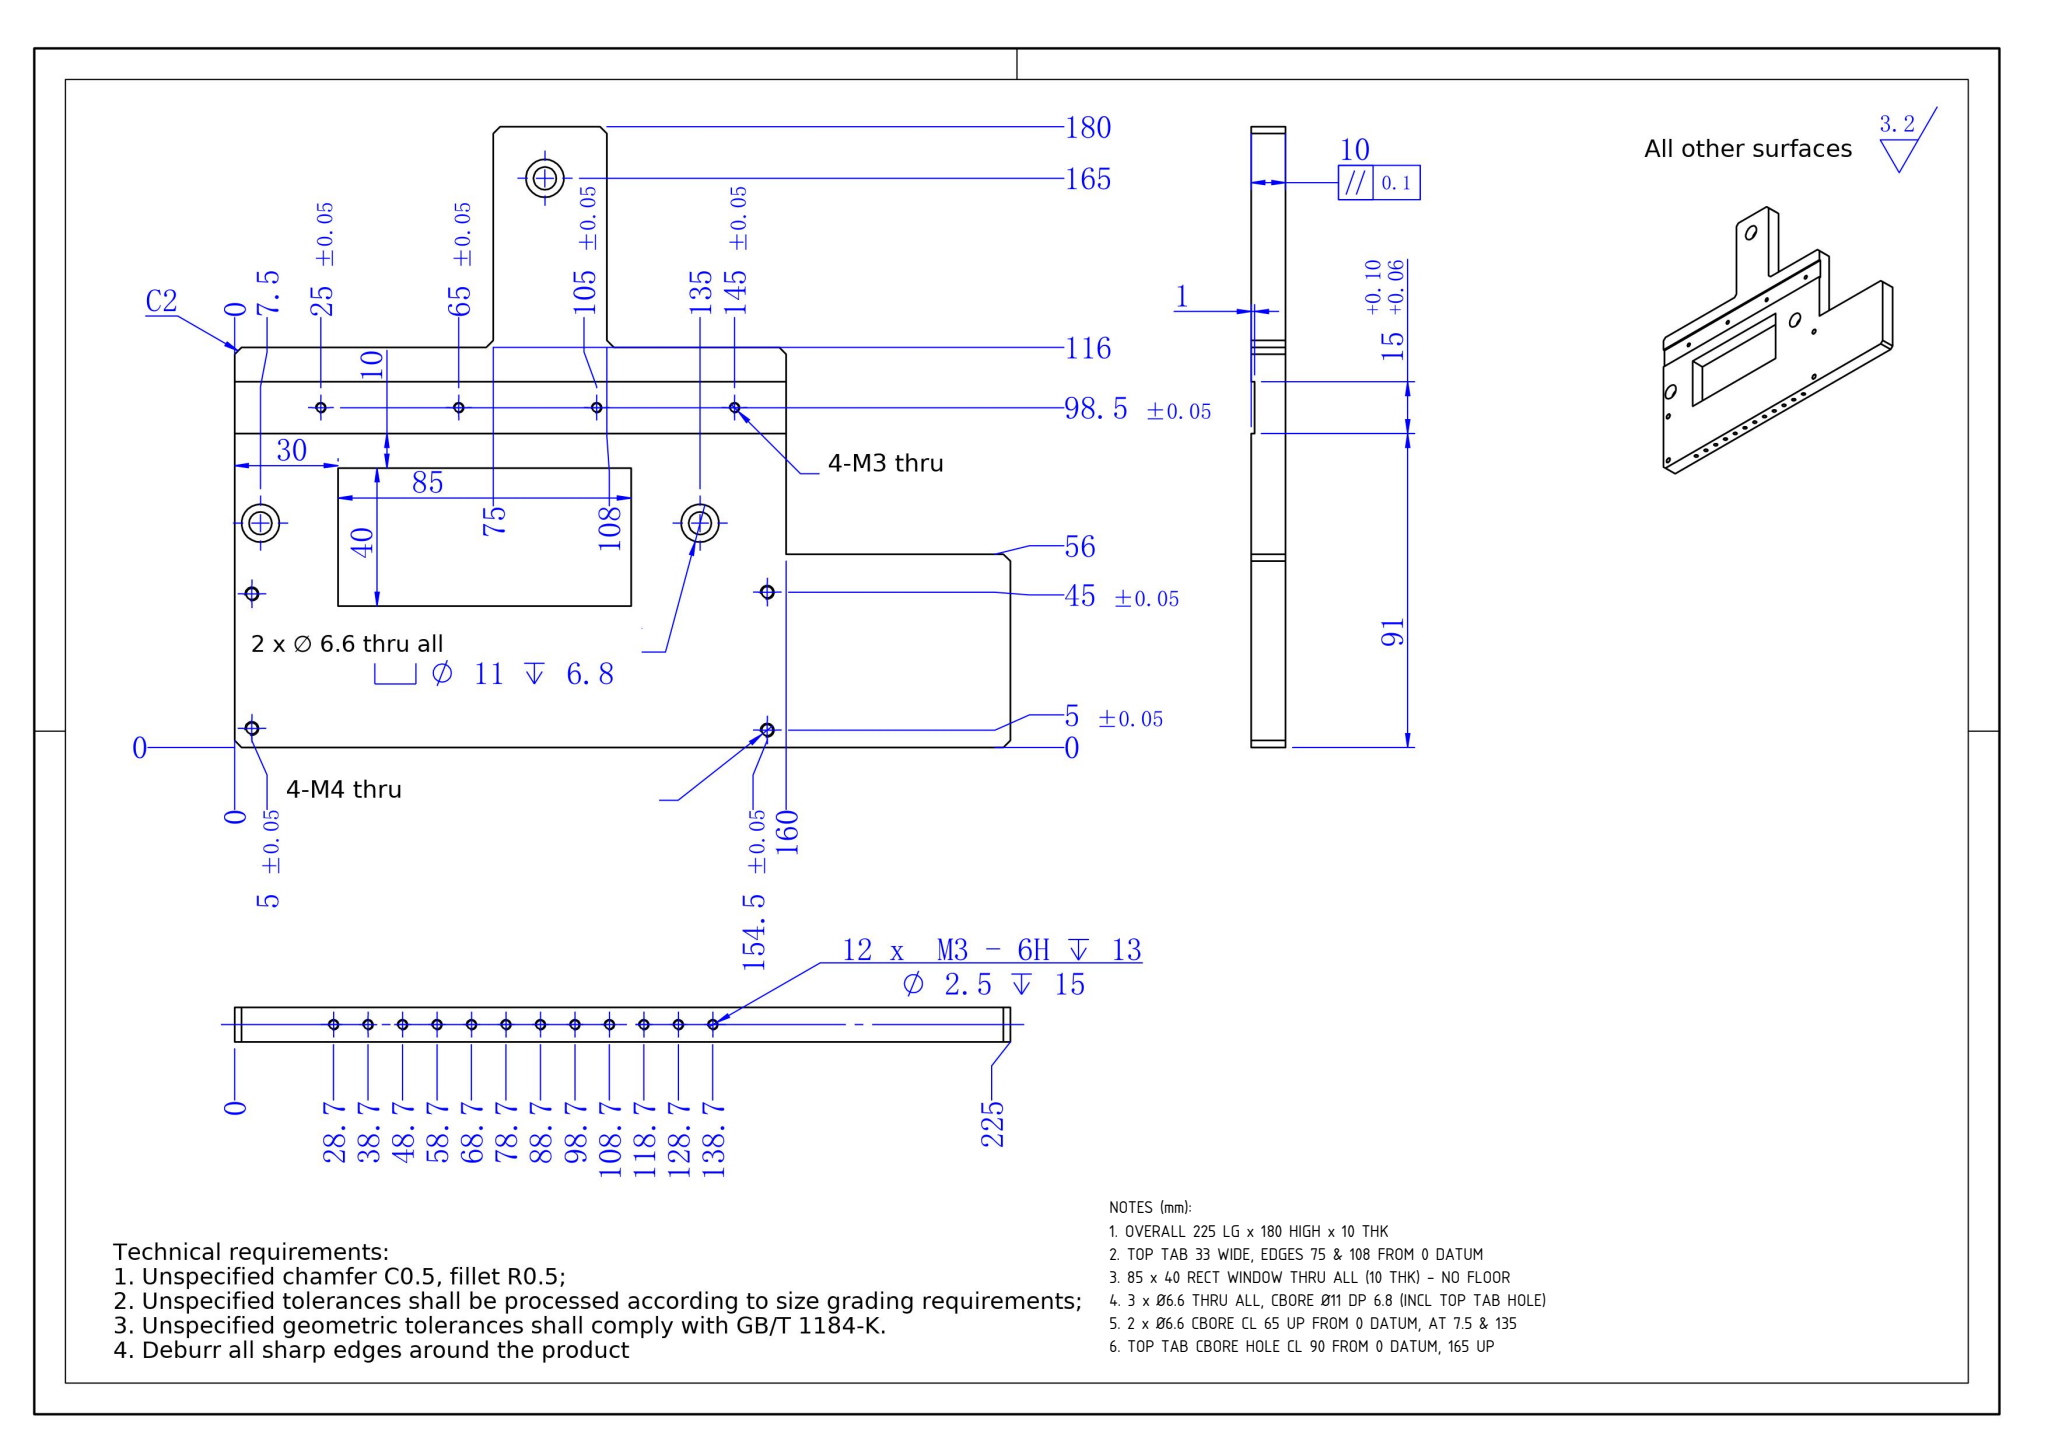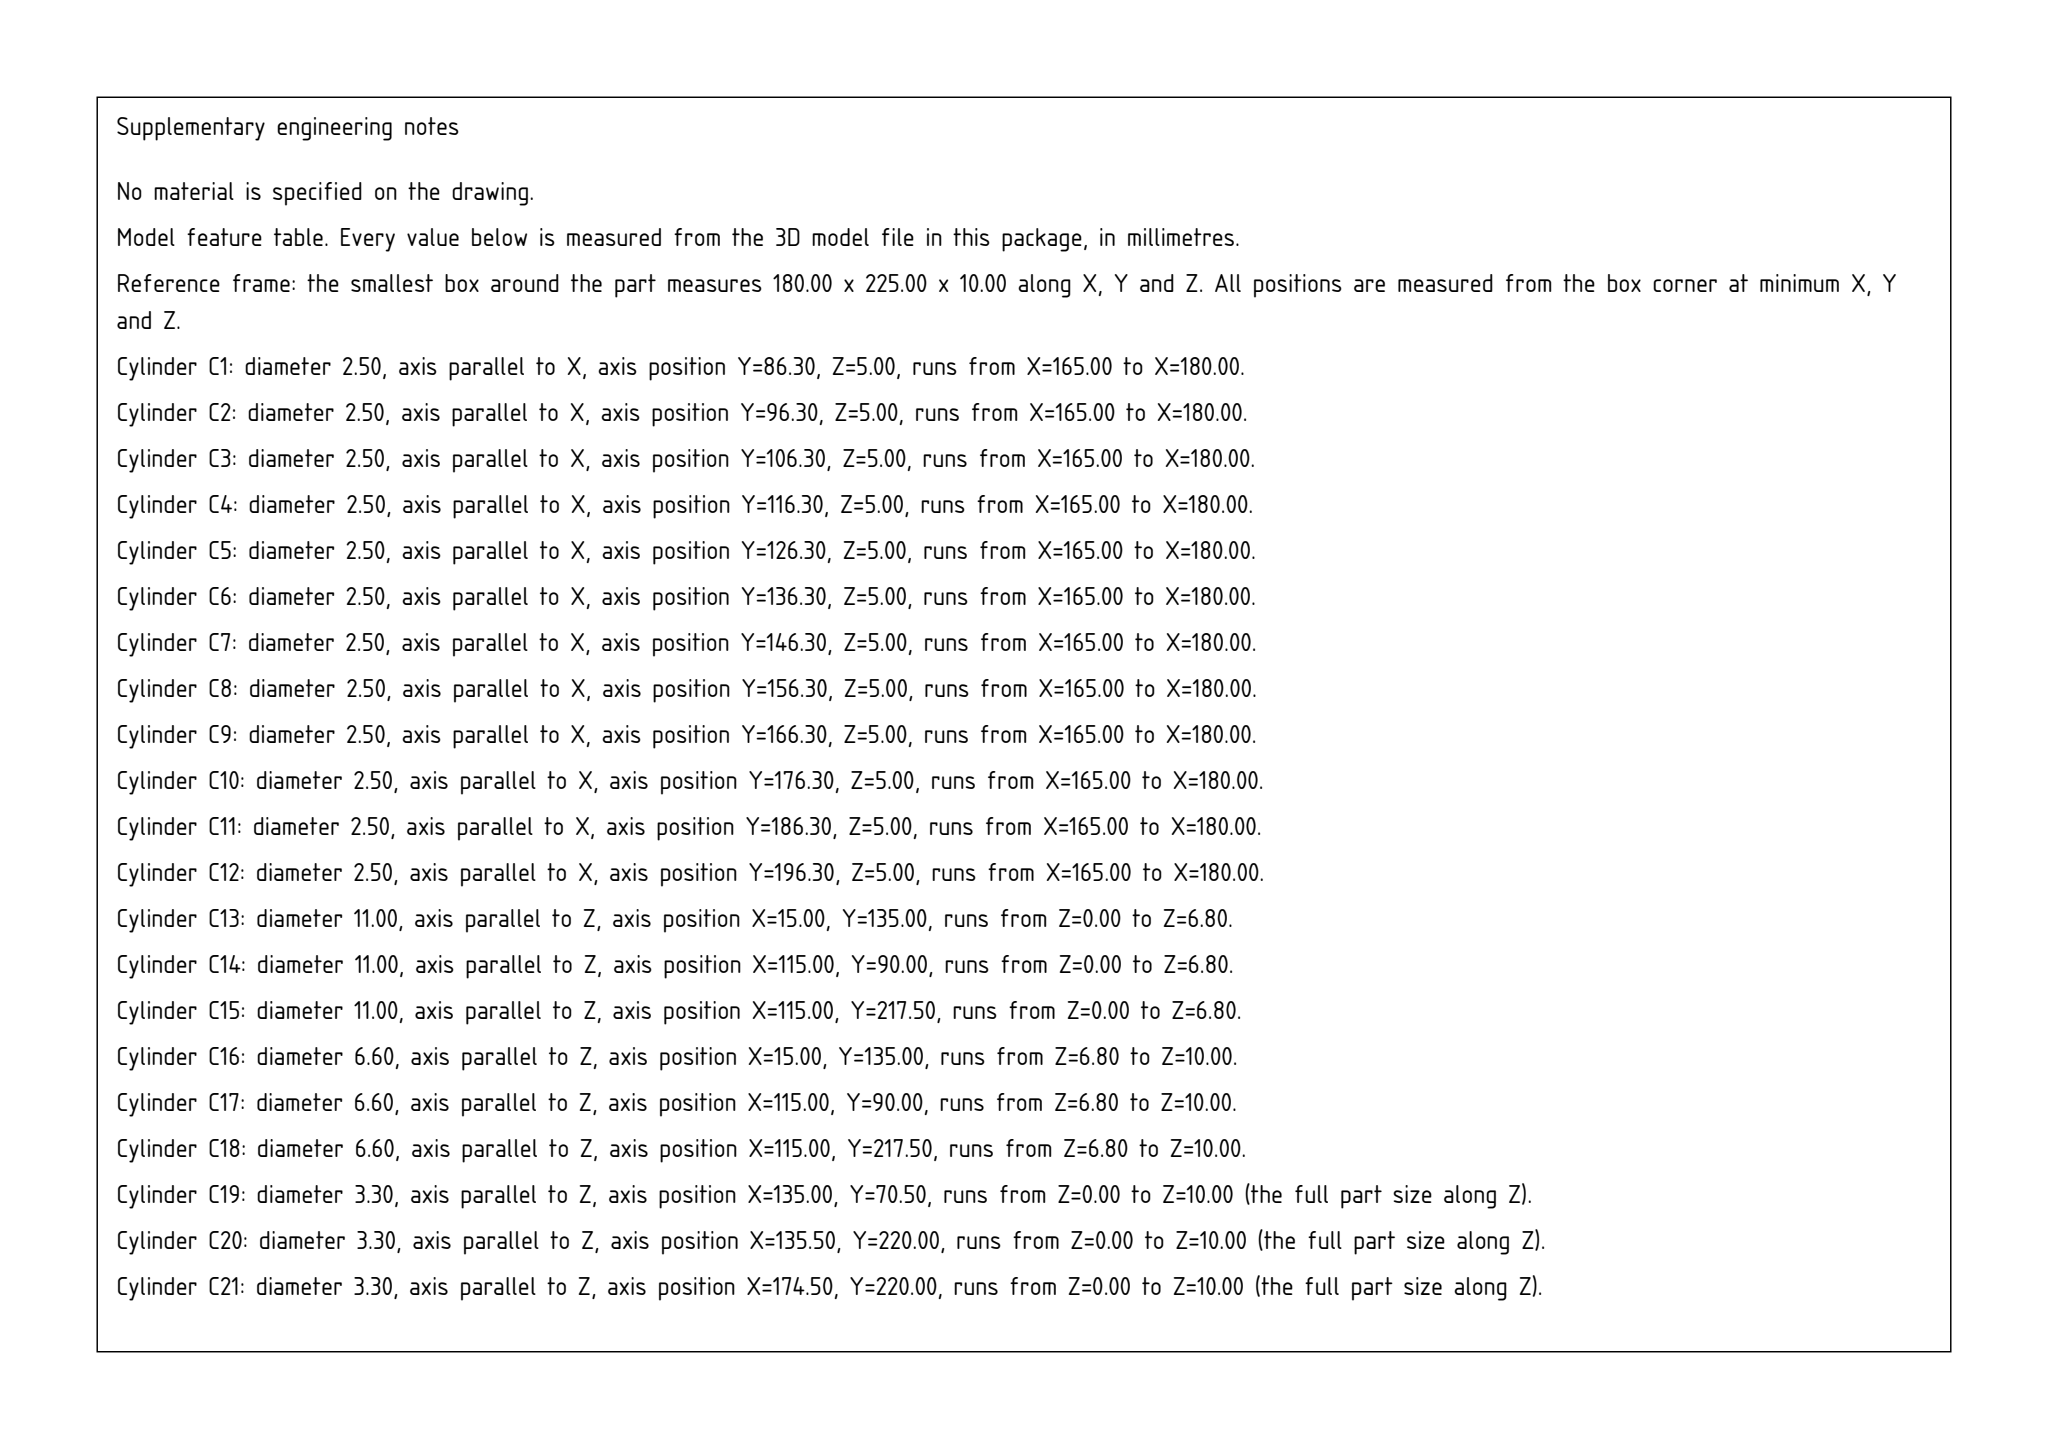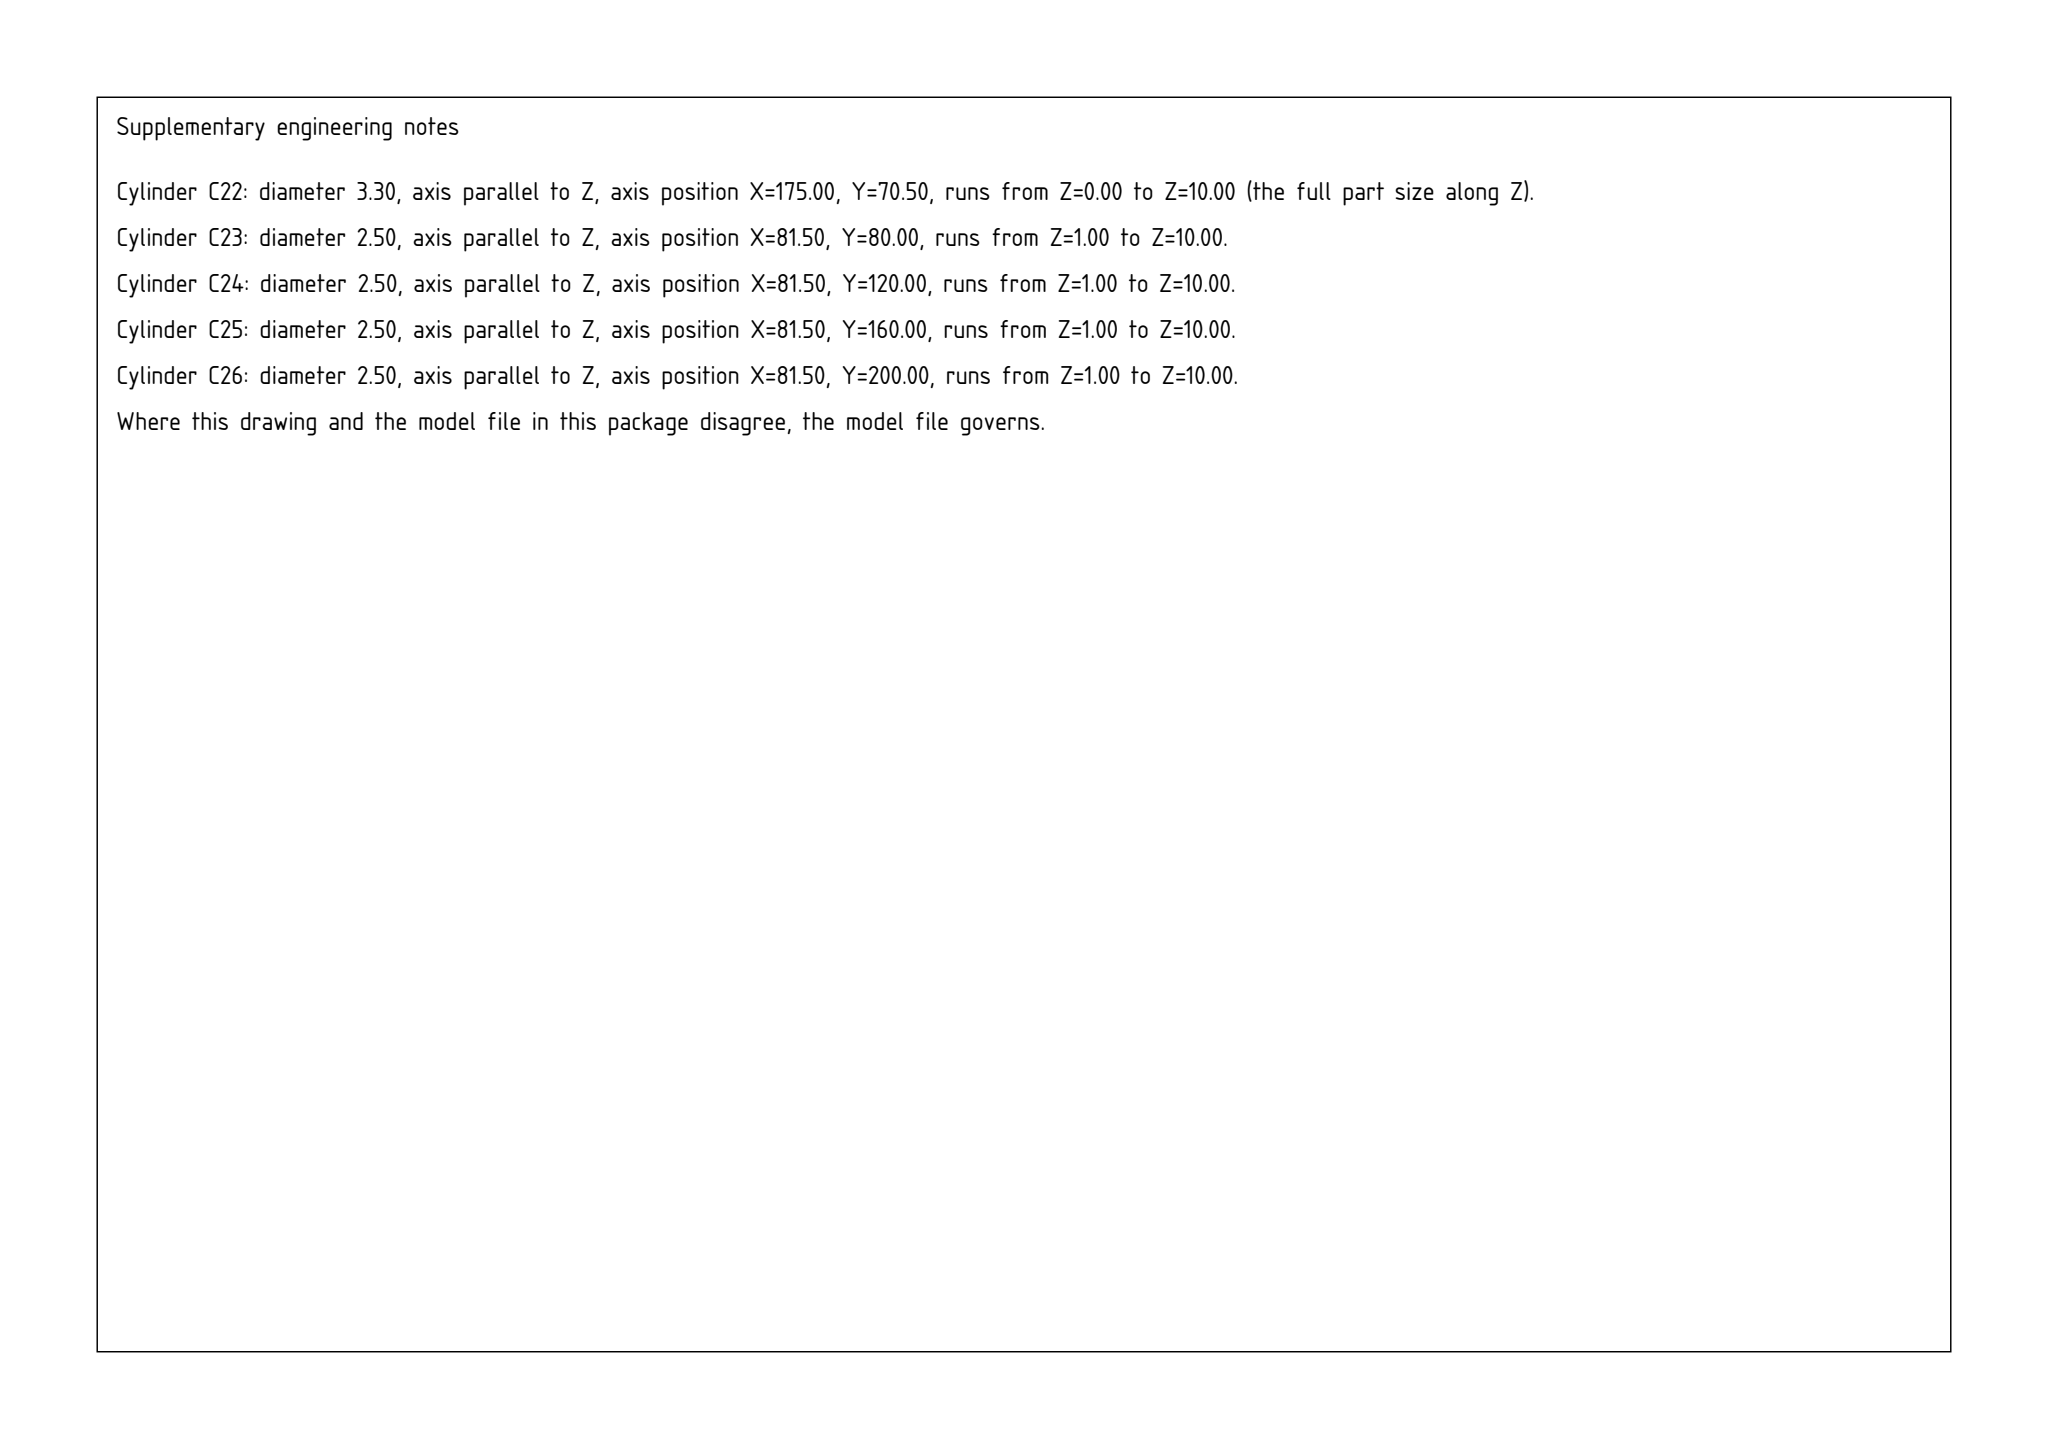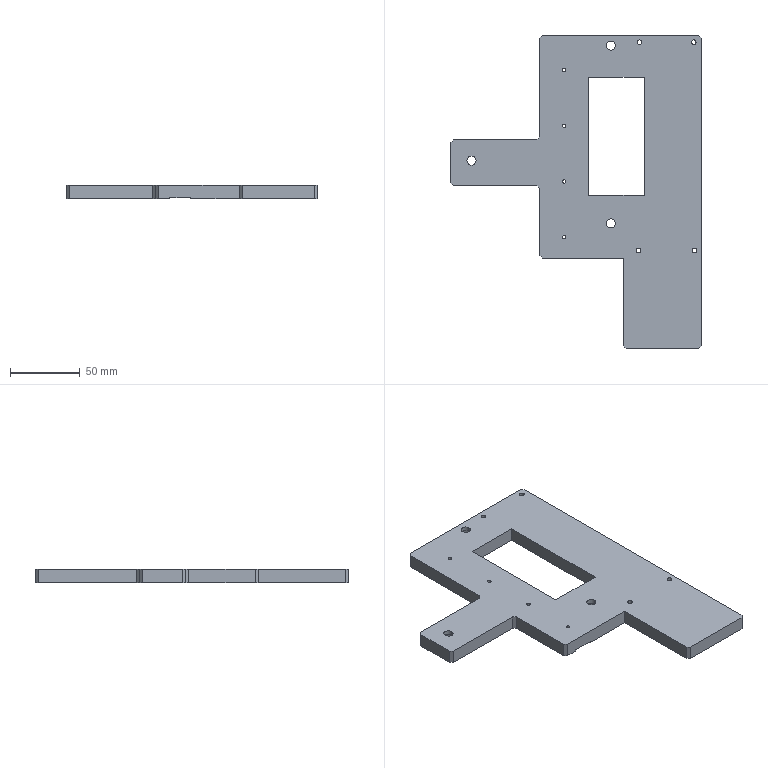Part | SolidWorks | mm | 1 solid | 108 faces | box 180 x 225 x 10 mm | volume 202936 mm3 | cylinder 52 | plane 32 | cone 24 | commonest cylinder face diameters 2.5 x32 3.3 x8 11 x6 6.6 x6
Drawing notes:
OVERALL 225 LG x 180 HIGH x 10 THK | from the solid: bbox_xyz 180 x 225 x 10; front view vert = 180-x, horiz = 225-y
TOP TAB 33 WIDE, EDGES 75 & 108 FROM 0 DATUM | from the solid: Y planes at 117 and 150 -> h=225-150=75, h=225-117=108; width 33
85 x 40 RECT WINDOW THRU ALL (10 THK) - NO FLOOR | from the solid: Window x99-139 (40) y110-195 (85); z planes only 0,1,6.8,10 so no pocket floor
3 x Ø6.6 THRU ALL, CBORE Ø11 DP 6.8 (INCL TOP TAB HOLE) | from the solid: Ø6.6 thru + Ø11 DP6.8 cyls at [15,135], [115,90], [115,217.5]
2 x Ø6.6 CBORE CL 65 UP FROM 0 DATUM, AT 7.5 & 135 | from the solid: Cyls at x=115 -> 180-115=65 up; y=217.5 -> h=7.5 and y=90 -> h=135
TOP TAB CBORE HOLE CL 90 FROM 0 DATUM, 165 UP | from the solid: Ø6.6/Ø11 DP6.8 cyl at [15,135] -> h=225-135=90, v=180-15=165
build123d program:
from build123d import *

# Parameters (mm, degrees)
SKETCH1_W                                          = 180
SKETCH1_H                                          = 230
BOSS_EXTRUDE1_DEPTH                                = 10
HOLE_SIZE_ACCORDING_TO_TYPE_OF_HEXAGON_D           = 6.6
HOLE_SIZE_ACCORDING_TO_TYPE_OF_HEXAGON_CBORE_D     = 11
HOLE_SIZE_ACCORDING_TO_TYPE_OF_HEXAGON_CBORE_DEPTH = 6.8
SKETCH12_W                                         = 64
SKETCH12_H                                         = 145
CUT_EXTRUDE1_DEPTH                                 = 10
CHAMFER2_SIZE                                      = 2
HOLE_SIZE_ACCORDING_TO_TYPE_OF_HEX_2_D             = 6.6
HOLE_SIZE_ACCORDING_TO_TYPE_OF_HEX_2_CBORE_D       = 11
HOLE_SIZE_ACCORDING_TO_TYPE_OF_HEX_2_CBORE_DEPTH   = 6.8
SKETCH20_W                                         = 109.885
SKETCH20_H                                         = 81.118
CUT_EXTRUDE5_DEPTH                                 = 10
CHAMFER3_SIZE                                      = 2
SKETCH21_W                                         = 96.639
SKETCH21_H                                         = 103.671
CUT_EXTRUDE6_DEPTH                                 = 10
SKETCH22_W                                         = 15
SKETCH22_H                                         = 1
CUT_EXTRUDE7_DEPTH                                 = 242.039
M3_TAPPED_HOLE1_D                                  = 2.5
M4_TAPPED_HOLE1_D                                  = 3.3
LPATTERN1_COUNT                                    = 12
LPATTERN1_PITCH                                    = 10
M5_TAPPED_HOLE1_D                                  = 4.2
SKETCH33_W                                         = 56
SKETCH33_H                                         = 65
BOSS_EXTRUDE2_DEPTH                                = 10
SKETCH34_W                                         = 76
SKETCH34_H                                         = 70
CUT_EXTRUDE8_DEPTH                                 = 293.233
CHAMFER4_SIZE                                      = 2
SKETCH35_W                                         = 40
SKETCH35_H                                         = 85
CUT_EXTRUDE9_DEPTH                                 = 10


with BuildPart() as part:
    # Sketch1 → Boss-Extrude1 (new body)
    with BuildSketch(Plane.XY):
        with Locations((90, 115)):
            Rectangle(SKETCH1_W, SKETCH1_H)
    extrude(amount=BOSS_EXTRUDE1_DEPTH)

    # Hole Size _According to_ Type of Hexagon (through all)
    with Locations(Plane(origin=(0, 0, 0), x_dir=(-1, 0, 0), z_dir=(0, 0, -1))):
        with Locations((-15, 70), (-115, 25)):
            CounterBoreHole(HOLE_SIZE_ACCORDING_TO_TYPE_OF_HEXAGON_D / 2, HOLE_SIZE_ACCORDING_TO_TYPE_OF_HEXAGON_CBORE_D / 2, HOLE_SIZE_ACCORDING_TO_TYPE_OF_HEXAGON_CBORE_DEPTH)

    # Sketch12 → Cut-Extrude1 (cut)
    with BuildSketch(Plane(origin=(0, 0, 0), x_dir=(-1, 0, 0), z_dir=(0, 0, -1))):
        with Locations((-32, 157.5)):
            Rectangle(SKETCH12_W, SKETCH12_H)
    extrude(amount=-CUT_EXTRUDE1_DEPTH, mode=Mode.SUBTRACT)

    # Chamfer2
    chamfer2_edges = [part.edges().sort_by_distance(p)[0] for p in [
        (0, 85, 5),
        (64, 85, 5),
    ]]
    chamfer(chamfer2_edges, length=CHAMFER2_SIZE)

    # Hole Size _According to_ Type of Hex 2 (through all)
    with Locations(Plane(origin=(0, 0, 0), x_dir=(-1, 0, 0), z_dir=(0, 0, -1))):
        with Locations((-115, 152.5)):
            CounterBoreHole(HOLE_SIZE_ACCORDING_TO_TYPE_OF_HEX_2_D / 2, HOLE_SIZE_ACCORDING_TO_TYPE_OF_HEX_2_CBORE_D / 2, HOLE_SIZE_ACCORDING_TO_TYPE_OF_HEX_2_CBORE_DEPTH)

    # Sketch20 → Cut-Extrude5 (cut)
    with BuildSketch(Plane(origin=(0, 0, 0), x_dir=(-1, 0, 0), z_dir=(0, 0, -1))):
        with Locations((-9.058, 11.441)):
            Rectangle(SKETCH20_W, SKETCH20_H)
    extrude(amount=-CUT_EXTRUDE5_DEPTH, mode=Mode.SUBTRACT)

    # Chamfer3
    chamfer3_edges = [part.edges().sort_by_distance(p)[0] for p in [
        (0, 52, 5),
        (64, 52, 5),
        (64, 0, 5),
    ]]
    chamfer(chamfer3_edges, length=CHAMFER3_SIZE)

    # Sketch21 → Cut-Extrude6 (cut)
    with BuildSketch(Plane(origin=(0, 0, 0), x_dir=(-1, 0, 0), z_dir=(0, 0, -1))):
        with Locations((-55.681, 211.835)):
            Rectangle(SKETCH21_W, SKETCH21_H)
    extrude(amount=-CUT_EXTRUDE6_DEPTH, mode=Mode.SUBTRACT)

    # Sketch22 → Cut-Extrude7 (cut, through all)
    with BuildSketch(Plane(origin=(0, 160, 0), x_dir=(1, 0, 0), z_dir=(0, 1, 0))):
        with Locations((81.5, -0.5)):
            Rectangle(SKETCH22_W, SKETCH22_H)
    extrude(amount=-CUT_EXTRUDE7_DEPTH, mode=Mode.SUBTRACT)

    # M3 Tapped Hole1 (through all)
    with Locations(Plane(origin=(0, 0, 0), x_dir=(-1, 0, 0), z_dir=(0, 0, -1))):
        with Locations((-81.5, 135), (-81.5, 95), (-81.5, 55), (-81.5, 15)):
            Hole(M3_TAPPED_HOLE1_D / 2)

    # M4 Tapped Hole1 (through all)
    with Locations(Plane(origin=(0, 0, 0), x_dir=(-1, 0, 0), z_dir=(0, 0, -1))):
        with Locations((-135.5, 155), (-174.5, 155), (-135, 5.5), (-175, 5.5)):
            Hole(M4_TAPPED_HOLE1_D / 2)

    # Sketch29 → M3 Tapped Hole2 (revolve, cut)
    with BuildSketch(Plane(origin=(180, 131.3, 5), x_dir=(0, 0, -1), z_dir=(0, 1, 0))):
        Polygon((0, 0), (0, 15.751), (1.25, 15), (1.25, 0), align=None)
    m3_tapped_hole2 = revolve(axis=Axis((186.35, 131.3, 5), (-1, 0, 0)), mode=Mode.SUBTRACT)

    # LPattern1: M3 Tapped Hole2 ×12
    with Locations(*[(0, -i * LPATTERN1_PITCH, 0) for i in range(1, LPATTERN1_COUNT)]):
        add(m3_tapped_hole2, mode=Mode.SUBTRACT)

    # M5 Tapped Hole1 (through all)
    with Locations(Plane(origin=(0, 0, 0), x_dir=(-1, 0, 0), z_dir=(0, 0, -1))):
        with Locations((-124, 200), (-146, 200)):
            Hole(M5_TAPPED_HOLE1_D / 2)

    # Sketch33 → Boss-Extrude2 (add)
    with BuildSketch(Plane(origin=(0, 0, 0), x_dir=(-1, 0, 0), z_dir=(0, 0, -1))):
        with Locations((-152, -32.5)):
            Rectangle(SKETCH33_W, SKETCH33_H)
    extrude(amount=-BOSS_EXTRUDE2_DEPTH)

    # Sketch34 → Cut-Extrude8 (cut, through all)
    with BuildSketch(Plane(origin=(0, 0, 0), x_dir=(-1, 0, 0), z_dir=(0, 0, -1))):
        with Locations((-142, 195)):
            Rectangle(SKETCH34_W, SKETCH34_H)
    extrude(amount=-CUT_EXTRUDE8_DEPTH, mode=Mode.SUBTRACT)

    # Chamfer4
    chamfer4_edges = [part.edges().sort_by_distance(p)[0] for p in [
        (64, 160, 5),
        (180, -65, 5),
        (124, -65, 5),
        (180, 160, 5),
    ]]
    chamfer(chamfer4_edges, length=CHAMFER4_SIZE)

    # Sketch35 → Cut-Extrude9 (cut)
    with BuildSketch(Plane(origin=(0, 0, 0), x_dir=(-1, 0, 0), z_dir=(0, 0, -1))):
        with Locations((-119, 87.5)):
            Rectangle(SKETCH35_W, SKETCH35_H)
    extrude(amount=-CUT_EXTRUDE9_DEPTH, mode=Mode.SUBTRACT)


solid = part.part